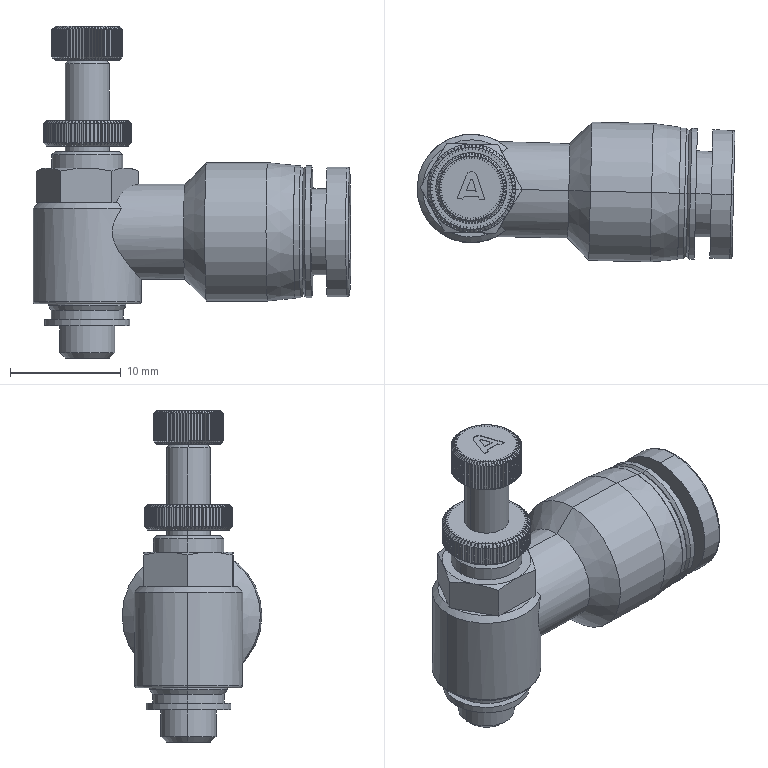Component | SolidWorks | PurchasedPart_ThrottleValvePSL6M5ABy-1 | 1 solid | 836 faces | box 28.73 x 12.63 x 30 mm | volume 2559 mm3 | plane 334 | cone 312 | cylinder 181 | torus 8 | sphere 1 | commonest cylinder face diameters 6.4 x74 8 x72 4 x6 11.9 x4 12.5 x2 7.8 x2 11.7 x2 6 x2